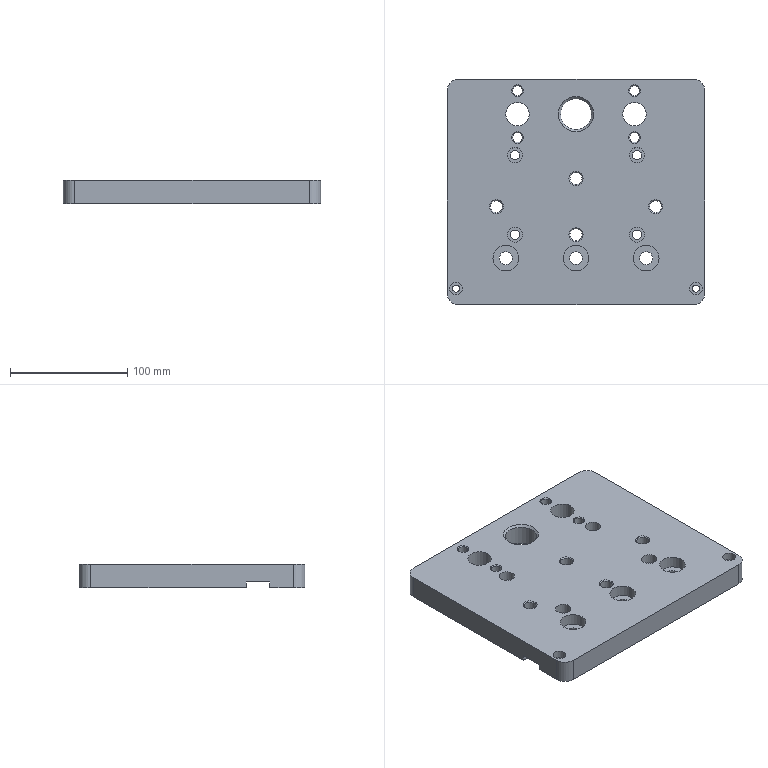Component | NX | CYL_FIX_PLATE | 1 solid | 70 faces | volume 768496 mm3 | cylinder 33 | plane 19 | cone 18 | commonest cylinder face diameters 20 x6 11 x5 8.5 x4 8 x4 13 x4 10.3 x4 22 x3 6 x2